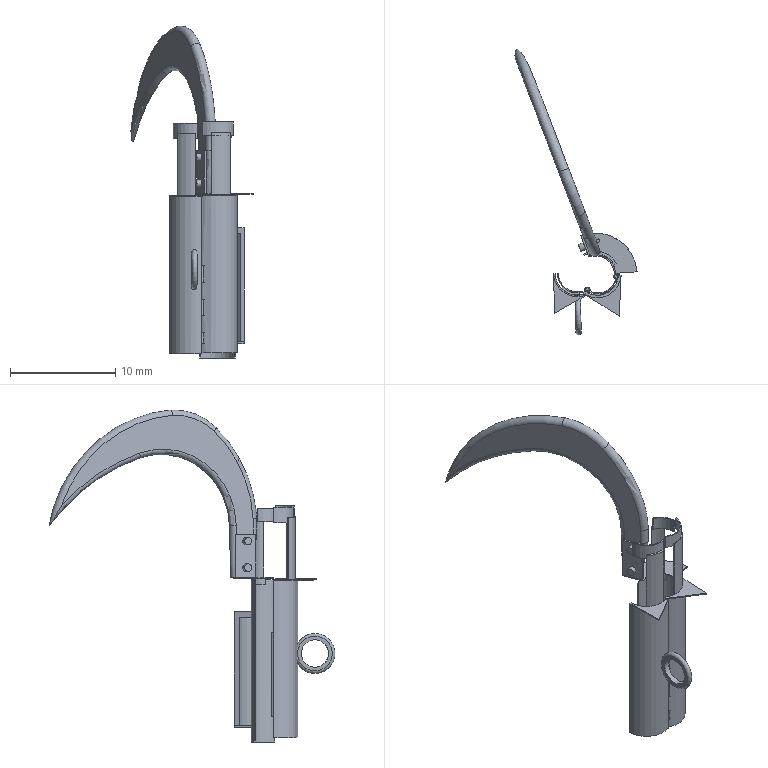Assembly | NX | mm | 8 component files | 21 solids | 211 faces | box 11.6 x 27.1 x 31.51 mm | volume 145 mm3 | plane 127 | cylinder 74 | torus 8 | cone 2 | commonest cylinder face diameters 0.4 x15 0.5 x14 3.8 x8 1.1 x6 4.5 x4 3.6 x4 4.2 x3 4.197 x3
Bill of materials:
unnamed part 1 | 1 |  | Long, thin, curved sheet-like body. From the side it looks like a narrow vertical bar with a stepped upper section. From above it is an arc-shaped sector. A small torus-like ring sticks out from one side, and there are three small knuckle-like tabs along one edge.
unnamed part 2 | 2 |  | Stepped cylindrical pin. A short, larger-diameter cylindrical head is joined coaxially to a longer, smaller-diameter cylindrical shank with flat ends.
unnamed part 3 | 1 |  | Elongated curved sheet-like body. From the side it looks like a stepped bar: a wider lower section, a narrower middle neck and a short wider cap at the top. From above it is a curved arc with small circular ring-like features at both ends. Small notches or tabs run along one edge of the lower section.
unnamed part 4 | 1 |  | Thin, crescent- or horn-shaped curved plate. It tapers from a wider rounded end to a pointed tip and has rounded edges. Two small through-holes sit near the wider end.
unnamed part 5 | 2 |  | Plain, slender solid cylindrical rod with flat ends and a constant diameter.
unnamed part 6 | 1 |  | Composite curved body. From above it is a wide arc-shaped sector with a small protruding stub at one end and a small ring at the other. From the side it is a stepped column with a narrow upper post. Other visible features: a rectangular tab with two holes, a rectangular open frame or window along one side, several small tabs along one edge, and thin curved flange plates.
Mates:
1. fix | HANDLE_SIDE 1 component
2. concentric | MIDDLE_PART 1 edge | HANDLE_SIDE 1 edge
3. concentric | FINGER_HOLDER 1 edge | MIDDLE_PART 1 edge
4. concentric | CUTTING_BLADE 1 edge | HANDLE_SIDE 1 edge
5. concentric | PIN 2 edge | HANDLE_SIDE 1 edge
6. concentric | PIN 1 edge | MIDDLE_PART 1 edge
7. concentric | BOLT 2 edge | HANDLE_SIDE 1 edge
8. concentric | BOLT 1 edge | HANDLE_SIDE 1 edge